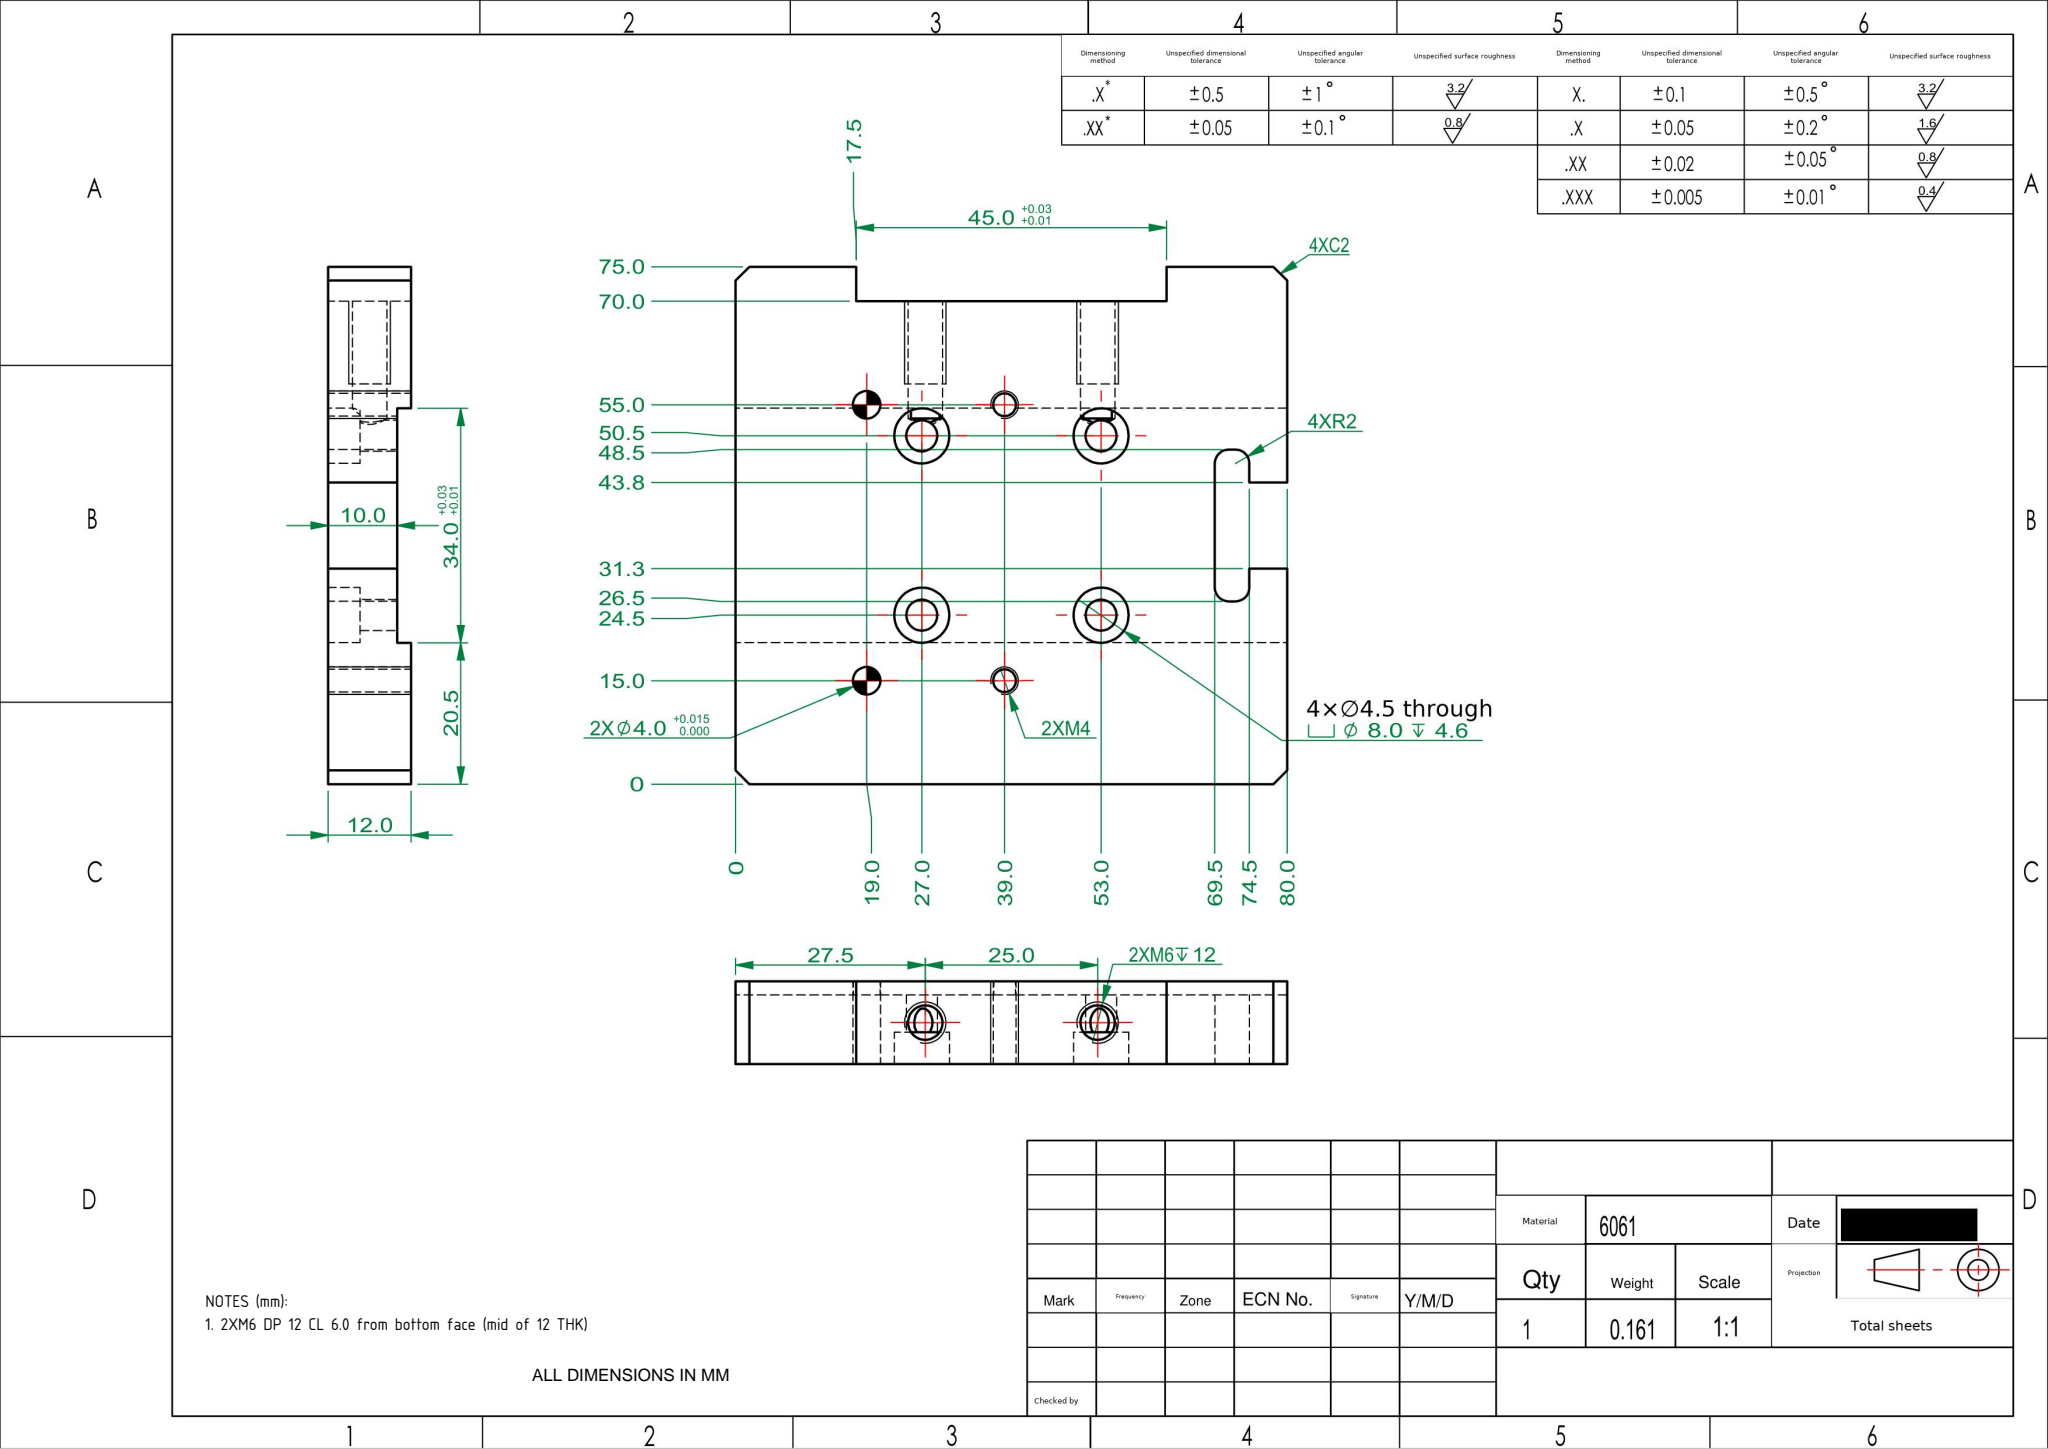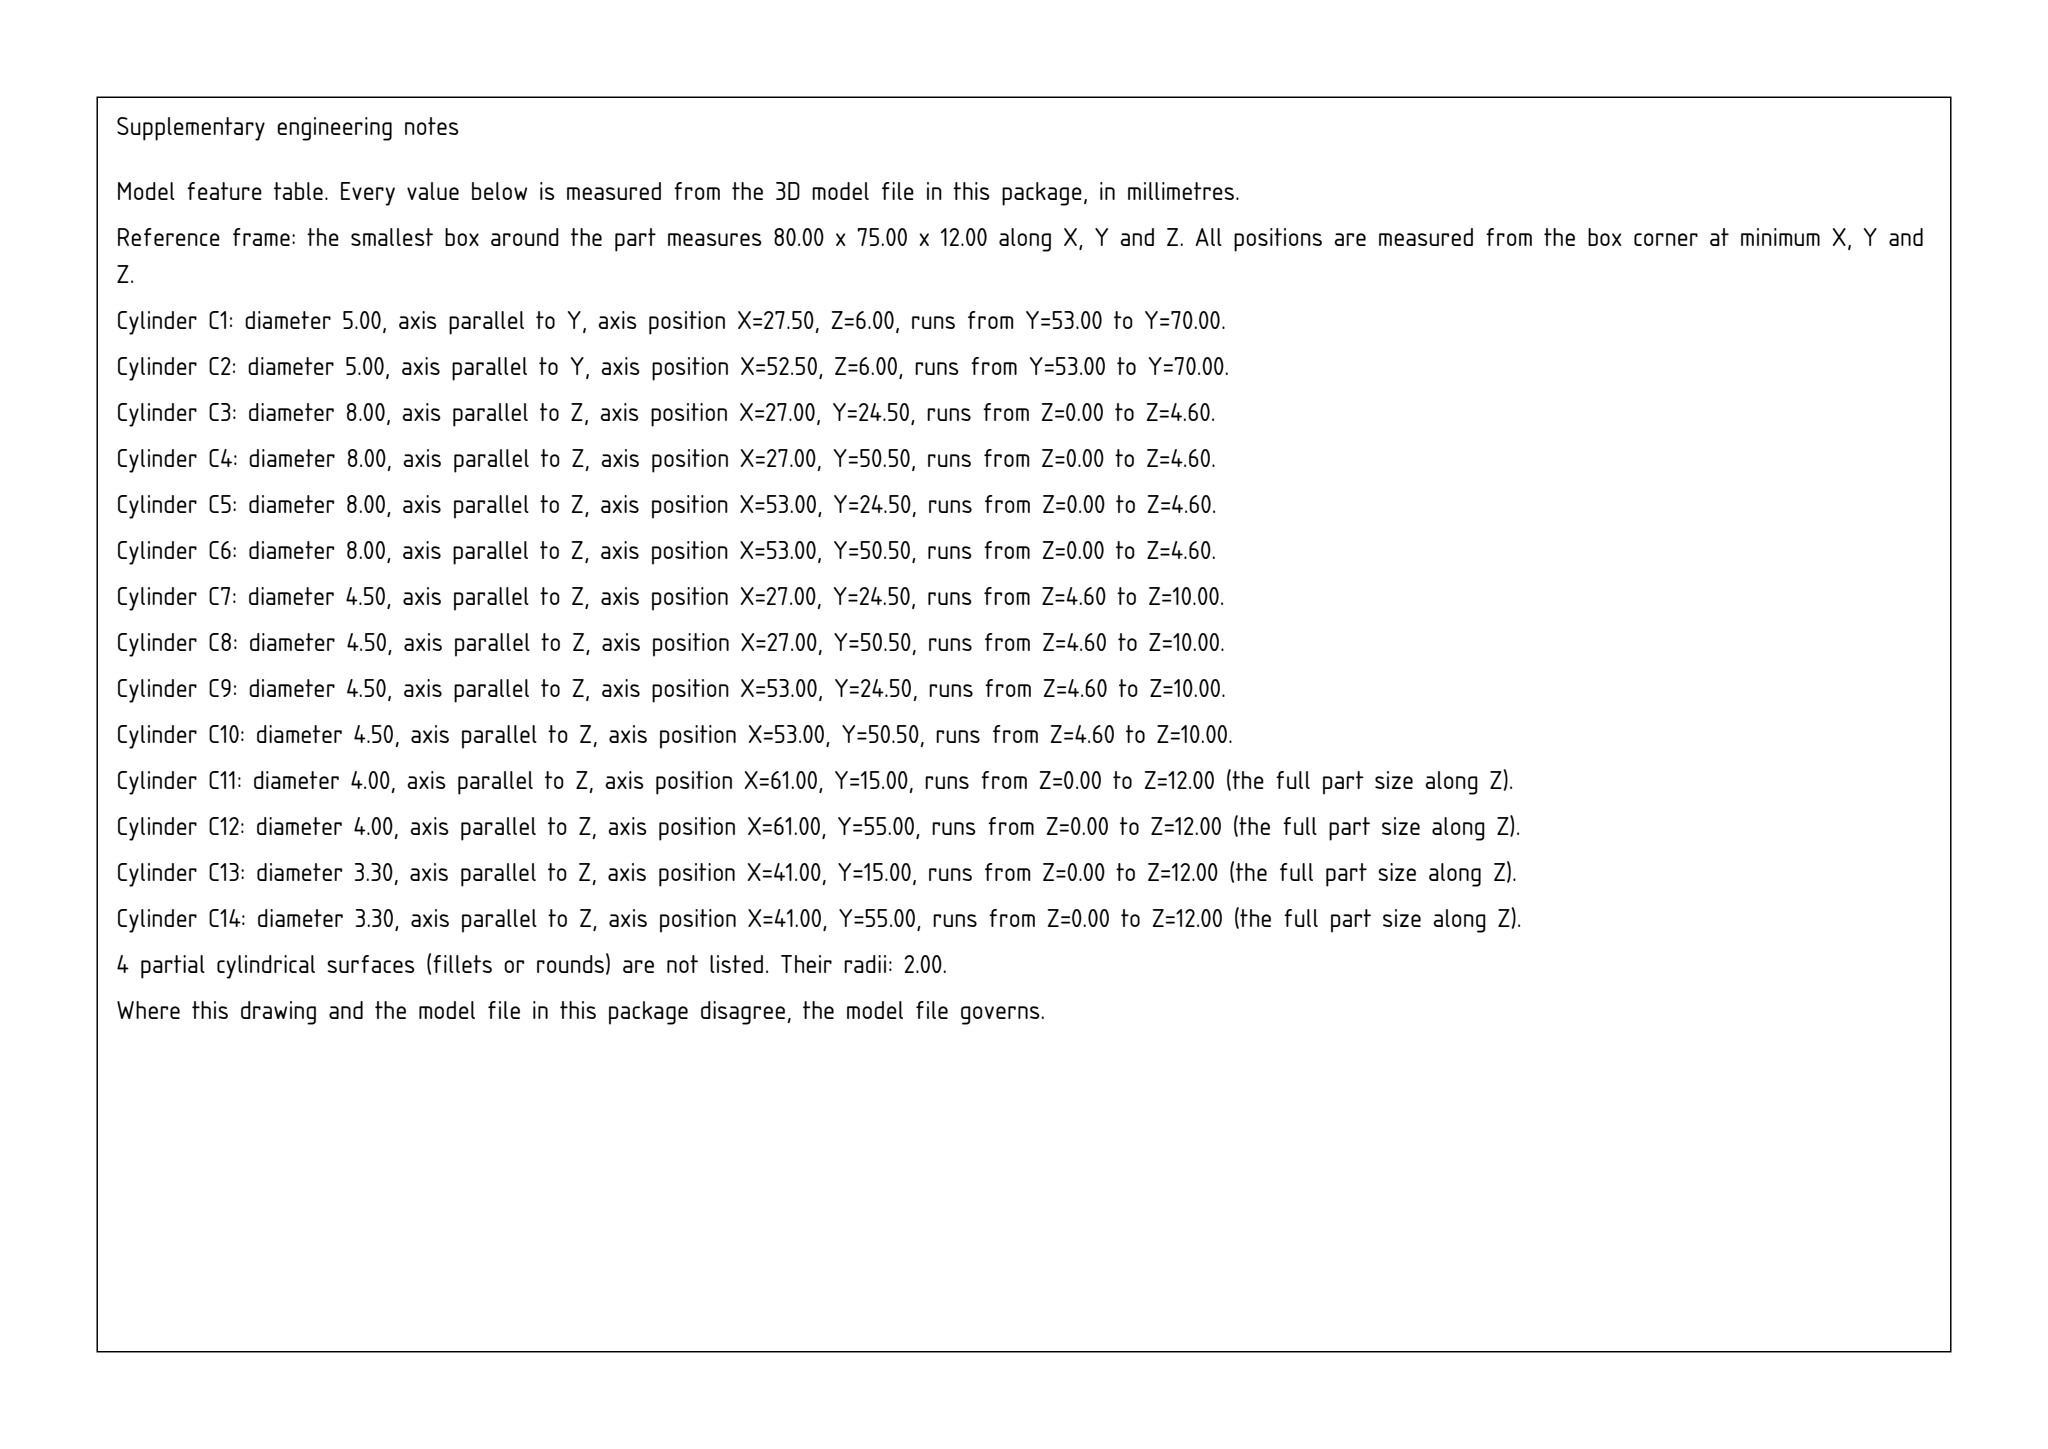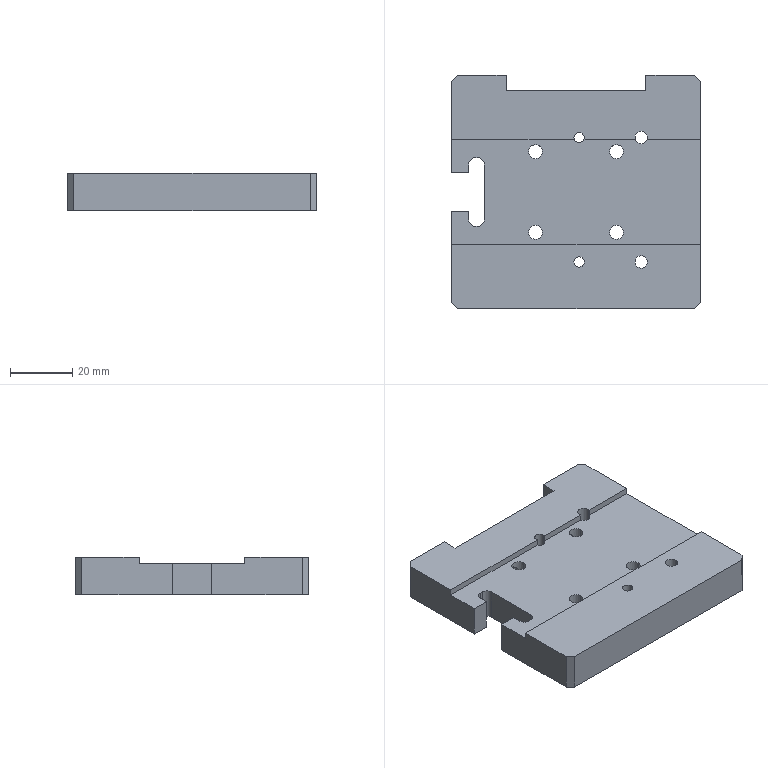Part | SolidWorks | mm | 1 solid | 68 faces | box 80 x 75 x 12 mm | volume 59580 mm3 | cylinder 32 | plane 32 | cone 4 | commonest cylinder face diameters 8 x8 4.5 x8 4 x8 5 x4 3.3 x4
Drawing notes:
2XM6 DP 12 CL 6.0 from bottom face (mid of 12 THK) | from the solid: cylinders dia 5.0 axis y at [27.5,-,6.0] and [52.5,-,6.0]; bbox Z=12.0
build123d program:
from build123d import *

# Parameters (mm, degrees)
SKETCH1_W                                         = 80
SKETCH1_H                                         = 75
BOSS_EXTRUDE1_DEPTH                               = 12
M4_TAPPED_HOLE1_D                                 = 3.3
SIZE_MM_DOWEL_PIN_HOLE1_D                         = 4
SKETCH5_W                                         = 80
SKETCH5_H                                         = 34
CUT_EXTRUDE1_DEPTH                                = 2
HOLE_SIZE_ACCORDING_TO_HEXAGON_SOCKET_D           = 4.5
HOLE_SIZE_ACCORDING_TO_HEXAGON_SOCKET_CBORE_D     = 8
HOLE_SIZE_ACCORDING_TO_HEXAGON_SOCKET_CBORE_DEPTH = 4.6
SKETCH8_W                                         = 16
SKETCH8_H                                         = 12.5
CUT_EXTRUDE2_DEPTH                                = 28
SKETCH9_W                                         = 5
SKETCH9_H                                         = 22
CUT_EXTRUDE3_DEPTH                                = 28
SKETCH10_W                                        = 45
SKETCH10_H                                        = 10
CUT_EXTRUDE4_DEPTH                                = 33
CHAMFER1_SIZE                                     = 2
M6_TAPPED_HOLE1_D                                 = 5
M6_TAPPED_HOLE1_DEPTH                             = 17
M6_TAPPED_HOLE1_TIP                               = 1.502
FILLET1_R                                         = 2


with BuildPart() as part:
    # Sketch1 → Boss-Extrude1 (new body)
    with BuildSketch(Plane.XY):
        Rectangle(SKETCH1_W, SKETCH1_H)
    extrude(amount=BOSS_EXTRUDE1_DEPTH)

    # M4 Tapped Hole1 (through all)
    with Locations(Plane(origin=(1, 17.5, 12), x_dir=(1, 0, 0), z_dir=(0, 0, 1))):
        with Locations((0, 0), (0, -40)):
            Hole(M4_TAPPED_HOLE1_D / 2)

    # Size mm Dowel Pin Hole1 (through all)
    with Locations(Plane(origin=(21, 17.5, 12), x_dir=(1, 0, 0), z_dir=(0, 0, 1))):
        with Locations((0, 0), (0, -40)):
            Hole(SIZE_MM_DOWEL_PIN_HOLE1_D / 2)

    # Sketch5 → Cut-Extrude1 (cut)
    with BuildSketch(Plane.XY.offset(12)):
        Rectangle(SKETCH5_W, SKETCH5_H)
    extrude(amount=-CUT_EXTRUDE1_DEPTH, mode=Mode.SUBTRACT)

    # Hole Size _ according to_ Hexagon Socket (through all)
    with Locations(Plane(origin=(13, 13, 0), x_dir=(-1, 0, 0), z_dir=(0, 0, -1))):
        with Locations((0, 0), (26, 0), (26, -26), (0, -26)):
            CounterBoreHole(HOLE_SIZE_ACCORDING_TO_HEXAGON_SOCKET_D / 2, HOLE_SIZE_ACCORDING_TO_HEXAGON_SOCKET_CBORE_D / 2, HOLE_SIZE_ACCORDING_TO_HEXAGON_SOCKET_CBORE_DEPTH)

    # Sketch8 → Cut-Extrude2 (cut)
    with BuildSketch(Plane(origin=(0, 0, 0), x_dir=(-1, 0, 0), z_dir=(0, 0, -1))):
        with Locations((40, 0)):
            Rectangle(SKETCH8_W, SKETCH8_H)
    extrude(amount=-CUT_EXTRUDE2_DEPTH, mode=Mode.SUBTRACT)

    # Sketch9 → Cut-Extrude3 (cut)
    with BuildSketch(Plane(origin=(0, 0, 0), x_dir=(-1, 0, 0), z_dir=(0, 0, -1))):
        with Locations((32, 0)):
            Rectangle(SKETCH9_W, SKETCH9_H)
    extrude(amount=-CUT_EXTRUDE3_DEPTH, mode=Mode.SUBTRACT)

    # Sketch10 → Cut-Extrude4 (cut)
    with BuildSketch(Plane(origin=(0, 0, 0), x_dir=(-1, 0, 0), z_dir=(0, 0, -1))):
        with Locations((0, 37.5)):
            Rectangle(SKETCH10_W, SKETCH10_H)
    extrude(amount=-CUT_EXTRUDE4_DEPTH, mode=Mode.SUBTRACT)

    # Chamfer1
    chamfer1_edges = [part.edges().sort_by_distance(p)[0] for p in [
        (40, -37.5, 6),
        (-40, -37.5, 6),
        (-40, 37.5, 6),
        (40, 37.5, 6),
    ]]
    chamfer(chamfer1_edges, length=CHAMFER1_SIZE)

    # M6 Tapped Hole1
    with Locations(Plane(origin=(-12.5, 32.5, 6), x_dir=(0, 0, 1), z_dir=(0, 1, 0))):
        with Locations((0, 0), (0, 25)):
            Hole(M6_TAPPED_HOLE1_D / 2, depth=M6_TAPPED_HOLE1_DEPTH)
            with Locations((0, 0, -(M6_TAPPED_HOLE1_DEPTH + M6_TAPPED_HOLE1_TIP / 2))):  # 118° drill point
                Cone(0, M6_TAPPED_HOLE1_D / 2, M6_TAPPED_HOLE1_TIP, mode=Mode.SUBTRACT)

    # Fillet1
    fillet1_edges = [part.edges().sort_by_distance(p)[0] for p in [
        (-34.5, 11, 5),
        (-34.5, -11, 5),
        (-29.5, -11, 5),
        (-29.5, 11, 5),
    ]]
    fillet(fillet1_edges, radius=FILLET1_R)


solid = part.part